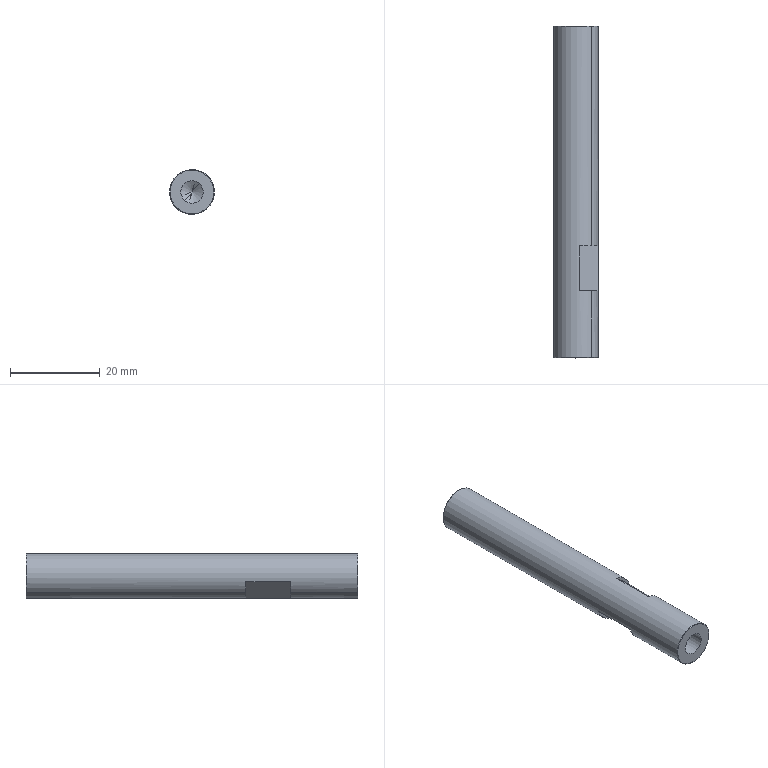Component | SolidWorks | F12529-M5105-2 | 1 solid | 22 faces | box 10 x 74 x 10 mm | volume 5066 mm3 | cone 8 | plane 8 | cylinder 6 | commonest cylinder face diameters 5 x4 10 x2
build123d program:
from build123d import *

# Parameters (mm, degrees)
SKETCH1_R             = 5
EXTRUDE1_DEPTH        = 74
CHAMFER1_SIZE         = 0.1
M6_TAPPED_HOLE1_D     = 5
M6_TAPPED_HOLE1_DEPTH = 17
M6_TAPPED_HOLE1_TIP   = 1.502
M6_TAPPED_HOLE2_D     = 5
M6_TAPPED_HOLE2_DEPTH = 17
M6_TAPPED_HOLE2_TIP   = 1.502
CUT_EXTRUDE2_START    = 4.2
SKETCH6_W             = 12
SKETCH6_H             = 10
CUT_EXTRUDE2_DEPTH    = 10


with BuildPart() as part:
    # Sketch1 → Extrude1 (new body)
    with BuildSketch(Plane(origin=(0, 0, 0), x_dir=(1, 0, 0), z_dir=(0, 1, 0))):
        with Locations(Location((0, 0, 0), (0, 0, 270))):
            Circle(SKETCH1_R)
    extrude(amount=EXTRUDE1_DEPTH)

    # Chamfer1
    chamfer1_edges = [part.edges().sort_by_distance(p)[0] for p in [
        (0, 0, -5),
        (0, 74, -5),
    ]]
    chamfer(chamfer1_edges, length=CHAMFER1_SIZE)

    # M6 Tapped Hole1
    with Locations(Plane(origin=(0, 74, 0), x_dir=(-1, 0, 0), z_dir=(0, 1, 0))):
        with Locations((0, 0)):
            Hole(M6_TAPPED_HOLE1_D / 2, depth=M6_TAPPED_HOLE1_DEPTH)
            with Locations((0, 0, -(M6_TAPPED_HOLE1_DEPTH + M6_TAPPED_HOLE1_TIP / 2))):  # 118° drill point
                Cone(0, M6_TAPPED_HOLE1_D / 2, M6_TAPPED_HOLE1_TIP, mode=Mode.SUBTRACT)

    # M6 Tapped Hole2
    with Locations(Plane.XZ):
        with Locations((0, 0)):
            Hole(M6_TAPPED_HOLE2_D / 2, depth=M6_TAPPED_HOLE2_DEPTH)
            with Locations((0, 0, -(M6_TAPPED_HOLE2_DEPTH + M6_TAPPED_HOLE2_TIP / 2))):  # 118° drill point
                Cone(0, M6_TAPPED_HOLE2_D / 2, M6_TAPPED_HOLE2_TIP, mode=Mode.SUBTRACT)

    # Sketch6 → Cut-Extrude2 (cut)
    with BuildSketch(Plane.XY.offset(CUT_EXTRUDE2_START)):
        with Locations((0, 20)):
            Rectangle(SKETCH6_W, SKETCH6_H)
    cut_extrude2 = extrude(amount=CUT_EXTRUDE2_DEPTH, mode=Mode.SUBTRACT)

    # Mirror1: Cut-Extrude2 across plane
    add(cut_extrude2.mirror(Plane.XY), mode=Mode.SUBTRACT)


solid = part.part

# Placed as in the assembly
solid = solid.moved(Location((-37.5, 201, -10), (180, -42.85, 180)))
STEP:
#1=COLOUR_RGB('',0.7922,0.8196,0.9333);
#2=FILL_AREA_STYLE_COLOUR('',#1);
#3=FILL_AREA_STYLE('',(#2));
#4=SURFACE_STYLE_FILL_AREA(#3);
#5=SURFACE_SIDE_STYLE('',(#4));
#6=SURFACE_STYLE_USAGE(.BOTH.,#5);
#7=PRESENTATION_STYLE_ASSIGNMENT((#6));
#8=CARTESIAN_POINT('',(-1.476,8.642,-0.3937));
#9=VERTEX_POINT('',#8);
#10=CARTESIAN_POINT('',(-1.543,8.583,-0.4659));
#11=VERTEX_POINT('',#10);
#12=CARTESIAN_POINT('',(-1.543,8.583,-0.4659));
#13=DIRECTION('',(-0.5829,-0.515,-0.6284));
#14=VECTOR('',#13,39.37);
#15=LINE('',#12,#14);
#16=EDGE_CURVE('',#9,#11,#15,.T.);
#17=ORIENTED_EDGE('',*,*,#16,.F.);
#18=CARTESIAN_POINT('',(-1.409,8.583,-0.3215));
#19=VERTEX_POINT('',#18);
#20=CARTESIAN_POINT('',(-1.409,8.583,-0.3215));
#21=DIRECTION('',(0.5829,-0.515,0.6284));
#22=VECTOR('',#21,39.37);
#23=LINE('',#20,#22);
#24=EDGE_CURVE('',#9,#19,#23,.T.);
#25=ORIENTED_EDGE('',*,*,#24,.T.);
#26=CARTESIAN_POINT('',(-1.476,8.583,-0.3937));
#27=DIRECTION('',(0.,-1.,0.));
#28=DIRECTION('',(-0.6801,0.,-0.7331));
#29=AXIS2_PLACEMENT_3D('',#26,#27,#28);
#30=CIRCLE('',#29,0.09843);
#31=EDGE_CURVE('',#19,#11,#30,.T.);
#32=ORIENTED_EDGE('',*,*,#31,.T.);
#33=EDGE_LOOP('',(#17,#25,#32));
#34=FACE_OUTER_BOUND('',#33,.T.);
#35=CARTESIAN_POINT('',(-1.476,8.583,-0.3937));
#36=DIRECTION('',(0.,-1.,0.));
#37=DIRECTION('',(-0.6801,0.,-0.7331));
#38=AXIS2_PLACEMENT_3D('',#35,#36,#37);
#39=CONICAL_SURFACE('',#38,0.09843,1.03);
#40=ADVANCED_FACE('',(#34),#39,.F.);
#41=ORIENTED_EDGE('',*,*,#31,.F.);
#42=CARTESIAN_POINT('',(-1.409,7.913,-0.3215));
#43=VERTEX_POINT('',#42);
#44=CARTESIAN_POINT('',(-1.409,7.913,-0.3215));
#45=DIRECTION('',(0.,-1.,0.));
#46=VECTOR('',#45,39.37);
#47=LINE('',#44,#46);
#48=EDGE_CURVE('',#19,#43,#47,.T.);
#49=ORIENTED_EDGE('',*,*,#48,.T.);
#50=CARTESIAN_POINT('',(-1.543,7.913,-0.4659));
#51=VERTEX_POINT('',#50);
#52=CARTESIAN_POINT('',(-1.476,7.913,-0.3937));
#53=DIRECTION('',(0.,-1.,0.));
#54=DIRECTION('',(-0.6801,0.,-0.7331));
#55=AXIS2_PLACEMENT_3D('',#52,#53,#54);
#56=CIRCLE('',#55,0.09843);
#57=EDGE_CURVE('',#43,#51,#56,.T.);
#58=ORIENTED_EDGE('',*,*,#57,.T.);
#59=CARTESIAN_POINT('',(-1.543,7.913,-0.4659));
#60=DIRECTION('',(0.,-1.,0.));
#61=VECTOR('',#60,39.37);
#62=LINE('',#59,#61);
#63=EDGE_CURVE('',#11,#51,#62,.T.);
#64=ORIENTED_EDGE('',*,*,#63,.F.);
#65=EDGE_LOOP('',(#41,#49,#58,#64));
#66=FACE_OUTER_BOUND('',#65,.T.);
#67=CARTESIAN_POINT('',(-1.476,7.913,-0.3937));
#68=DIRECTION('',(0.,-1.,0.));
#69=DIRECTION('',(-0.6801,0.,-0.7331));
#70=AXIS2_PLACEMENT_3D('',#67,#68,#69);
#71=CYLINDRICAL_SURFACE('',#70,0.09843);
#72=ADVANCED_FACE('',(#66),#71,.F.);
#73=CARTESIAN_POINT('',(-1.476,10.098,-0.3937));
#74=VERTEX_POINT('',#73);
#75=CARTESIAN_POINT('',(-1.409,10.157,-0.3215));
#76=VERTEX_POINT('',#75);
#77=CARTESIAN_POINT('',(-1.409,10.157,-0.3215));
#78=DIRECTION('',(0.5829,0.515,0.6284));
#79=VECTOR('',#78,39.37);
#80=LINE('',#77,#79);
#81=EDGE_CURVE('',#74,#76,#80,.T.);
#82=ORIENTED_EDGE('',*,*,#81,.F.);
#83=CARTESIAN_POINT('',(-1.543,10.157,-0.4659));
#84=VERTEX_POINT('',#83);
#85=CARTESIAN_POINT('',(-1.543,10.157,-0.4659));
#86=DIRECTION('',(-0.5829,0.515,-0.6284));
#87=VECTOR('',#86,39.37);
#88=LINE('',#85,#87);
#89=EDGE_CURVE('',#74,#84,#88,.T.);
#90=ORIENTED_EDGE('',*,*,#89,.T.);
#91=CARTESIAN_POINT('',(-1.476,10.157,-0.3937));
#92=DIRECTION('',(0.,1.,0.));
#93=DIRECTION('',(0.6801,0.,0.7331));
#94=AXIS2_PLACEMENT_3D('',#91,#92,#93);
#95=CIRCLE('',#94,0.09843);
#96=EDGE_CURVE('',#84,#76,#95,.T.);
#97=ORIENTED_EDGE('',*,*,#96,.T.);
#98=EDGE_LOOP('',(#82,#90,#97));
#99=FACE_OUTER_BOUND('',#98,.T.);
#100=CARTESIAN_POINT('',(-1.476,10.157,-0.3937));
#101=DIRECTION('',(0.,1.,0.));
#102=DIRECTION('',(0.6801,0.,0.7331));
#103=AXIS2_PLACEMENT_3D('',#100,#101,#102);
#104=CONICAL_SURFACE('',#103,0.09843,1.03);
#105=ADVANCED_FACE('',(#99),#104,.F.);
#106=ORIENTED_EDGE('',*,*,#96,.F.);
#107=CARTESIAN_POINT('',(-1.543,10.827,-0.4659));
#108=VERTEX_POINT('',#107);
#109=CARTESIAN_POINT('',(-1.543,10.827,-0.4659));
#110=DIRECTION('',(0.,1.,0.));
#111=VECTOR('',#110,39.37);
#112=LINE('',#109,#111);
#113=EDGE_CURVE('',#84,#108,#112,.T.);
#114=ORIENTED_EDGE('',*,*,#113,.T.);
#115=CARTESIAN_POINT('',(-1.409,10.827,-0.3215));
#116=VERTEX_POINT('',#115);
#117=CARTESIAN_POINT('',(-1.476,10.827,-0.3937));
#118=DIRECTION('',(0.,1.,0.));
#119=DIRECTION('',(0.6801,0.,0.7331));
#120=AXIS2_PLACEMENT_3D('',#117,#118,#119);
#121=CIRCLE('',#120,0.09843);
#122=EDGE_CURVE('',#108,#116,#121,.T.);
#123=ORIENTED_EDGE('',*,*,#122,.T.);
#124=CARTESIAN_POINT('',(-1.409,10.827,-0.3215));
#125=DIRECTION('',(0.,1.,0.));
#126=VECTOR('',#125,39.37);
#127=LINE('',#124,#126);
#128=EDGE_CURVE('',#76,#116,#127,.T.);
#129=ORIENTED_EDGE('',*,*,#128,.F.);
#130=EDGE_LOOP('',(#106,#114,#123,#129));
#131=FACE_OUTER_BOUND('',#130,.T.);
#132=CARTESIAN_POINT('',(-1.476,10.827,-0.3937));
#133=DIRECTION('',(0.,1.,0.));
#134=DIRECTION('',(0.6801,0.,0.7331));
#135=AXIS2_PLACEMENT_3D('',#132,#133,#134);
#136=CYLINDRICAL_SURFACE('',#135,0.09843);
#137=ADVANCED_FACE('',(#131),#136,.F.);
#138=CARTESIAN_POINT('',(-1.345,10.827,-0.2523));
#139=VERTEX_POINT('',#138);
#140=CARTESIAN_POINT('',(-1.608,10.827,-0.5351));
#141=VERTEX_POINT('',#140);
#142=CARTESIAN_POINT('',(-1.476,10.827,-0.3937));
#143=DIRECTION('',(0.,1.,0.));
#144=DIRECTION('',(0.6801,0.,0.7331));
#145=AXIS2_PLACEMENT_3D('',#142,#143,#144);
#146=CIRCLE('',#145,0.1929);
#147=EDGE_CURVE('',#139,#141,#146,.T.);
#148=ORIENTED_EDGE('',*,*,#147,.F.);
#149=CARTESIAN_POINT('',(-1.343,10.823,-0.2494));
#150=VERTEX_POINT('',#149);
#151=CARTESIAN_POINT('',(-1.345,10.827,-0.2523));
#152=DIRECTION('',(0.4809,-0.7071,0.5184));
#153=VECTOR('',#152,39.37);
#154=LINE('',#151,#153);
#155=EDGE_CURVE('',#139,#150,#154,.T.);
#156=ORIENTED_EDGE('',*,*,#155,.T.);
#157=CARTESIAN_POINT('',(-1.61,10.823,-0.538));
#158=VERTEX_POINT('',#157);
#159=CARTESIAN_POINT('',(-1.476,10.823,-0.3937));
#160=DIRECTION('',(0.,-1.,0.));
#161=DIRECTION('',(0.6801,0.,0.7331));
#162=AXIS2_PLACEMENT_3D('',#159,#160,#161);
#163=CIRCLE('',#162,0.1969);
#164=EDGE_CURVE('',#158,#150,#163,.T.);
#165=ORIENTED_EDGE('',*,*,#164,.F.);
#166=CARTESIAN_POINT('',(-1.608,10.827,-0.5351));
#167=DIRECTION('',(-0.4809,-0.7071,-0.5184));
#168=VECTOR('',#167,39.37);
#169=LINE('',#166,#168);
#170=EDGE_CURVE('',#141,#158,#169,.T.);
#171=ORIENTED_EDGE('',*,*,#170,.F.);
#172=EDGE_LOOP('',(#148,#156,#165,#171));
#173=FACE_OUTER_BOUND('',#172,.T.);
#174=CARTESIAN_POINT('',(-1.476,10.827,-0.3937));
#175=DIRECTION('',(0.,-1.,0.));
#176=DIRECTION('',(-0.6801,0.,-0.7331));
#177=AXIS2_PLACEMENT_3D('',#174,#175,#176);
#178=CONICAL_SURFACE('',#177,0.1929,0.7854);
#179=ADVANCED_FACE('',(#173),#178,.T.);
#180=CARTESIAN_POINT('',(-1.608,7.913,-0.5351));
#181=VERTEX_POINT('',#180);
#182=CARTESIAN_POINT('',(-1.345,7.913,-0.2523));
#183=VERTEX_POINT('',#182);
#184=CARTESIAN_POINT('',(-1.476,7.913,-0.3937));
#185=DIRECTION('',(0.,-1.,0.));
#186=DIRECTION('',(0.6801,0.,0.7331));
#187=AXIS2_PLACEMENT_3D('',#184,#185,#186);
#188=CIRCLE('',#187,0.1929);
#189=EDGE_CURVE('',#181,#183,#188,.T.);
#190=ORIENTED_EDGE('',*,*,#189,.F.);
#191=CARTESIAN_POINT('',(-1.61,7.917,-0.538));
#192=VERTEX_POINT('',#191);
#193=CARTESIAN_POINT('',(-1.61,7.917,-0.538));
#194=DIRECTION('',(-0.4809,0.7071,-0.5184));
#195=VECTOR('',#194,39.37);
#196=LINE('',#193,#195);
#197=EDGE_CURVE('',#181,#192,#196,.T.);
#198=ORIENTED_EDGE('',*,*,#197,.T.);
#199=CARTESIAN_POINT('',(-1.343,7.917,-0.2494));
#200=VERTEX_POINT('',#199);
#201=CARTESIAN_POINT('',(-1.476,7.917,-0.3937));
#202=DIRECTION('',(0.,1.,0.));
#203=DIRECTION('',(0.6801,0.,0.7331));
#204=AXIS2_PLACEMENT_3D('',#201,#202,#203);
#205=CIRCLE('',#204,0.1969);
#206=EDGE_CURVE('',#200,#192,#205,.T.);
#207=ORIENTED_EDGE('',*,*,#206,.F.);
#208=CARTESIAN_POINT('',(-1.343,7.917,-0.2494));
#209=DIRECTION('',(0.4809,0.7071,0.5184));
#210=VECTOR('',#209,39.37);
#211=LINE('',#208,#210);
#212=EDGE_CURVE('',#183,#200,#211,.T.);
#213=ORIENTED_EDGE('',*,*,#212,.F.);
#214=EDGE_LOOP('',(#190,#198,#207,#213));
#215=FACE_OUTER_BOUND('',#214,.T.);
#216=CARTESIAN_POINT('',(-1.476,7.917,-0.3937));
#217=DIRECTION('',(0.,1.,0.));
#218=DIRECTION('',(0.6801,0.,0.7331));
#219=AXIS2_PLACEMENT_3D('',#216,#217,#218);
#220=CONICAL_SURFACE('',#219,0.1969,0.7854);
#221=ADVANCED_FACE('',(#215),#220,.T.);
#222=ORIENTED_EDGE('',*,*,#164,.T.);
#223=CARTESIAN_POINT('',(-1.343,8.898,-0.2494));
#224=VERTEX_POINT('',#223);
#225=CARTESIAN_POINT('',(-1.343,10.827,-0.2494));
#226=DIRECTION('',(0.,-1.,0.));
#227=VECTOR('',#226,39.37);
#228=LINE('',#225,#227);
#229=EDGE_CURVE('',#150,#224,#228,.T.);
#230=ORIENTED_EDGE('',*,*,#229,.T.);
#231=CARTESIAN_POINT('',(-1.286,8.898,-0.3451));
#232=VERTEX_POINT('',#231);
#233=CARTESIAN_POINT('',(-1.476,8.898,-0.3937));
#234=DIRECTION('',(0.,-1.,0.));
#235=DIRECTION('',(-0.6801,0.,-0.7331));
#236=AXIS2_PLACEMENT_3D('',#233,#234,#235);
#237=CIRCLE('',#236,0.1969);
#238=EDGE_CURVE('',#232,#224,#237,.T.);
#239=ORIENTED_EDGE('',*,*,#238,.F.);
#240=CARTESIAN_POINT('',(-1.286,8.504,-0.3451));
#241=VERTEX_POINT('',#240);
#242=CARTESIAN_POINT('',(-1.286,10.827,-0.3451));
#243=DIRECTION('',(0.,1.,0.));
#244=VECTOR('',#243,39.37);
#245=LINE('',#242,#244);
#246=EDGE_CURVE('',#241,#232,#245,.T.);
#247=ORIENTED_EDGE('',*,*,#246,.F.);
#248=CARTESIAN_POINT('',(-1.343,8.504,-0.2494));
#249=VERTEX_POINT('',#248);
#250=CARTESIAN_POINT('',(-1.476,8.504,-0.3937));
#251=DIRECTION('',(0.,1.,0.));
#252=DIRECTION('',(0.6801,0.,0.7331));
#253=AXIS2_PLACEMENT_3D('',#250,#251,#252);
#254=CIRCLE('',#253,0.1969);
#255=EDGE_CURVE('',#249,#241,#254,.T.);
#256=ORIENTED_EDGE('',*,*,#255,.F.);
#257=CARTESIAN_POINT('',(-1.343,10.827,-0.2494));
#258=DIRECTION('',(0.,-1.,0.));
#259=VECTOR('',#258,39.37);
#260=LINE('',#257,#259);
#261=EDGE_CURVE('',#249,#200,#260,.T.);
#262=ORIENTED_EDGE('',*,*,#261,.T.);
#263=ORIENTED_EDGE('',*,*,#206,.T.);
#264=CARTESIAN_POINT('',(-1.61,8.504,-0.538));
#265=VERTEX_POINT('',#264);
#266=CARTESIAN_POINT('',(-1.61,10.827,-0.538));
#267=DIRECTION('',(0.,-1.,0.));
#268=VECTOR('',#267,39.37);
#269=LINE('',#266,#268);
#270=EDGE_CURVE('',#265,#192,#269,.T.);
#271=ORIENTED_EDGE('',*,*,#270,.F.);
#272=CARTESIAN_POINT('',(-1.511,8.504,-0.5876));
#273=VERTEX_POINT('',#272);
#274=CARTESIAN_POINT('',(-1.476,8.504,-0.3937));
#275=DIRECTION('',(0.,-1.,0.));
#276=DIRECTION('',(-0.6801,0.,-0.7331));
#277=AXIS2_PLACEMENT_3D('',#274,#275,#276);
#278=CIRCLE('',#277,0.1969);
#279=EDGE_CURVE('',#265,#273,#278,.T.);
#280=ORIENTED_EDGE('',*,*,#279,.T.);
#281=CARTESIAN_POINT('',(-1.511,8.898,-0.5876));
#282=VERTEX_POINT('',#281);
#283=CARTESIAN_POINT('',(-1.511,10.827,-0.5876));
#284=DIRECTION('',(0.,-1.,0.));
#285=VECTOR('',#284,39.37);
#286=LINE('',#283,#285);
#287=EDGE_CURVE('',#282,#273,#286,.T.);
#288=ORIENTED_EDGE('',*,*,#287,.F.);
#289=CARTESIAN_POINT('',(-1.61,8.898,-0.538));
#290=VERTEX_POINT('',#289);
#291=CARTESIAN_POINT('',(-1.476,8.898,-0.3937));
#292=DIRECTION('',(0.,1.,0.));
#293=DIRECTION('',(0.6801,0.,0.7331));
#294=AXIS2_PLACEMENT_3D('',#291,#292,#293);
#295=CIRCLE('',#294,0.1969);
#296=EDGE_CURVE('',#282,#290,#295,.T.);
#297=ORIENTED_EDGE('',*,*,#296,.T.);
#298=CARTESIAN_POINT('',(-1.61,10.827,-0.538));
#299=DIRECTION('',(0.,-1.,0.));
#300=VECTOR('',#299,39.37);
#301=LINE('',#298,#300);
#302=EDGE_CURVE('',#158,#290,#301,.T.);
#303=ORIENTED_EDGE('',*,*,#302,.F.);
#304=EDGE_LOOP('',(#222,#230,#239,#247,#256,#262,#263,#271,#280,#288,#297,#303));
#305=FACE_OUTER_BOUND('',#304,.T.);
#306=CARTESIAN_POINT('',(-1.476,10.827,-0.3937));
#307=DIRECTION('',(0.,-1.,0.));
#308=DIRECTION('',(-0.6801,0.,-0.7331));
#309=AXIS2_PLACEMENT_3D('',#306,#307,#308);
#310=CYLINDRICAL_SURFACE('',#309,0.1969);
#311=ADVANCED_FACE('',(#305),#310,.T.);
#312=ORIENTED_EDGE('',*,*,#229,.F.);
#313=CARTESIAN_POINT('',(-1.476,10.823,-0.3937));
#314=DIRECTION('',(0.,-1.,0.));
#315=DIRECTION('',(0.6801,0.,0.7331));
#316=AXIS2_PLACEMENT_3D('',#313,#314,#315);
#317=CIRCLE('',#316,0.1969);
#318=EDGE_CURVE('',#150,#158,#317,.T.);
#319=ORIENTED_EDGE('',*,*,#318,.T.);
#320=ORIENTED_EDGE('',*,*,#302,.T.);
#321=CARTESIAN_POINT('',(-1.667,8.898,-0.4423));
#322=VERTEX_POINT('',#321);
#323=CARTESIAN_POINT('',(-1.476,8.898,-0.3937));
#324=DIRECTION('',(0.,1.,0.));
#325=DIRECTION('',(0.6801,0.,0.7331));
#326=AXIS2_PLACEMENT_3D('',#323,#324,#325);
#327=CIRCLE('',#326,0.1969);
#328=EDGE_CURVE('',#290,#322,#327,.T.);
#329=ORIENTED_EDGE('',*,*,#328,.T.);
#330=CARTESIAN_POINT('',(-1.667,8.504,-0.4423));
#331=VERTEX_POINT('',#330);
#332=CARTESIAN_POINT('',(-1.667,10.827,-0.4423));
#333=DIRECTION('',(0.,1.,0.));
#334=VECTOR('',#333,39.37);
#335=LINE('',#332,#334);
#336=EDGE_CURVE('',#331,#322,#335,.T.);
#337=ORIENTED_EDGE('',*,*,#336,.F.);
#338=CARTESIAN_POINT('',(-1.476,8.504,-0.3937));
#339=DIRECTION('',(0.,-1.,0.));
#340=DIRECTION('',(-0.6801,0.,-0.7331));
#341=AXIS2_PLACEMENT_3D('',#338,#339,#340);
#342=CIRCLE('',#341,0.1969);
#343=EDGE_CURVE('',#331,#265,#342,.T.);
#344=ORIENTED_EDGE('',*,*,#343,.T.);
#345=ORIENTED_EDGE('',*,*,#270,.T.);
#346=CARTESIAN_POINT('',(-1.476,7.917,-0.3937));
#347=DIRECTION('',(0.,1.,0.));
#348=DIRECTION('',(0.6801,0.,0.7331));
#349=AXIS2_PLACEMENT_3D('',#346,#347,#348);
#350=CIRCLE('',#349,0.1969);
#351=EDGE_CURVE('',#192,#200,#350,.T.);
#352=ORIENTED_EDGE('',*,*,#351,.T.);
#353=ORIENTED_EDGE('',*,*,#261,.F.);
#354=CARTESIAN_POINT('',(-1.442,8.504,-0.1998));
#355=VERTEX_POINT('',#354);
#356=CARTESIAN_POINT('',(-1.476,8.504,-0.3937));
#357=DIRECTION('',(0.,1.,0.));
#358=DIRECTION('',(0.6801,0.,0.7331));
#359=AXIS2_PLACEMENT_3D('',#356,#357,#358);
#360=CIRCLE('',#359,0.1969);
#361=EDGE_CURVE('',#355,#249,#360,.T.);
#362=ORIENTED_EDGE('',*,*,#361,.F.);
#363=CARTESIAN_POINT('',(-1.442,8.898,-0.1998));
#364=VERTEX_POINT('',#363);
#365=CARTESIAN_POINT('',(-1.442,10.827,-0.1998));
#366=DIRECTION('',(0.,-1.,0.));
#367=VECTOR('',#366,39.37);
#368=LINE('',#365,#367);
#369=EDGE_CURVE('',#364,#355,#368,.T.);
#370=ORIENTED_EDGE('',*,*,#369,.F.);
#371=CARTESIAN_POINT('',(-1.476,8.898,-0.3937));
#372=DIRECTION('',(0.,-1.,0.));
#373=DIRECTION('',(-0.6801,0.,-0.7331));
#374=AXIS2_PLACEMENT_3D('',#371,#372,#373);
#375=CIRCLE('',#374,0.1969);
#376=EDGE_CURVE('',#224,#364,#375,.T.);
#377=ORIENTED_EDGE('',*,*,#376,.F.);
#378=EDGE_LOOP('',(#312,#319,#320,#329,#337,#344,#345,#352,#353,#362,#370,#377));
#379=FACE_OUTER_BOUND('',#378,.T.);
#380=CARTESIAN_POINT('',(-1.476,10.827,-0.3937));
#381=DIRECTION('',(0.,-1.,0.));
#382=DIRECTION('',(-0.6801,0.,-0.7331));
#383=AXIS2_PLACEMENT_3D('',#380,#381,#382);
#384=CYLINDRICAL_SURFACE('',#383,0.1969);
#385=ADVANCED_FACE('',(#379),#384,.T.);
#386=CARTESIAN_POINT('',(-1.476,10.827,-0.3937));
#387=DIRECTION('',(0.,1.,0.));
#388=DIRECTION('',(0.6801,0.,0.7331));
#389=AXIS2_PLACEMENT_3D('',#386,#387,#388);
#390=CIRCLE('',#389,0.09843);
#391=EDGE_CURVE('',#116,#108,#390,.T.);
#392=ORIENTED_EDGE('',*,*,#391,.F.);
#393=ORIENTED_EDGE('',*,*,#122,.F.);
#394=EDGE_LOOP('',(#392,#393));
#395=FACE_BOUND('',#394,.T.);
#396=CARTESIAN_POINT('',(-1.476,10.827,-0.3937));
#397=DIRECTION('',(0.,1.,0.));
#398=DIRECTION('',(0.6801,0.,0.7331));
#399=AXIS2_PLACEMENT_3D('',#396,#397,#398);
#400=CIRCLE('',#399,0.1929);
#401=EDGE_CURVE('',#141,#139,#400,.T.);
#402=ORIENTED_EDGE('',*,*,#401,.T.);
#403=ORIENTED_EDGE('',*,*,#147,.T.);
#404=EDGE_LOOP('',(#402,#403));
#405=FACE_OUTER_BOUND('',#404,.T.);
#406=CARTESIAN_POINT('',(-1.476,10.827,-0.3937));
#407=DIRECTION('',(0.,1.,0.));
#408=DIRECTION('',(0.6801,0.,0.7331));
#409=AXIS2_PLACEMENT_3D('',#406,#407,#408);
#410=PLANE('',#409);
#411=ADVANCED_FACE('',(#395,#405),#410,.T.);
#412=CARTESIAN_POINT('',(-1.476,7.913,-0.3937));
#413=DIRECTION('',(0.,-1.,0.));
#414=DIRECTION('',(-0.6801,0.,-0.7331));
#415=AXIS2_PLACEMENT_3D('',#412,#413,#414);
#416=CIRCLE('',#415,0.09843);
#417=EDGE_CURVE('',#51,#43,#416,.T.);
#418=ORIENTED_EDGE('',*,*,#417,.F.);
#419=ORIENTED_EDGE('',*,*,#57,.F.);
#420=EDGE_LOOP('',(#418,#419));
#421=FACE_BOUND('',#420,.T.);
#422=CARTESIAN_POINT('',(-1.476,7.913,-0.3937));
#423=DIRECTION('',(0.,-1.,0.));
#424=DIRECTION('',(0.6801,0.,0.7331));
#425=AXIS2_PLACEMENT_3D('',#422,#423,#424);
#426=CIRCLE('',#425,0.1929);
#427=EDGE_CURVE('',#183,#181,#426,.T.);
#428=ORIENTED_EDGE('',*,*,#427,.T.);
#429=ORIENTED_EDGE('',*,*,#189,.T.);
#430=EDGE_LOOP('',(#428,#429));
#431=FACE_OUTER_BOUND('',#430,.T.);
#432=CARTESIAN_POINT('',(-1.476,7.913,-0.3937));
#433=DIRECTION('',(0.,1.,0.));
#434=DIRECTION('',(0.6801,0.,0.7331));
#435=AXIS2_PLACEMENT_3D('',#432,#433,#434);
#436=PLANE('',#435);
#437=ADVANCED_FACE('',(#421,#431),#436,.F.);
#438=ORIENTED_EDGE('',*,*,#197,.F.);
#439=ORIENTED_EDGE('',*,*,#427,.F.);
#440=ORIENTED_EDGE('',*,*,#212,.T.);
#441=ORIENTED_EDGE('',*,*,#351,.F.);
#442=EDGE_LOOP('',(#438,#439,#440,#441));
#443=FACE_OUTER_BOUND('',#442,.T.);
#444=CARTESIAN_POINT('',(-1.476,7.917,-0.3937));
#445=DIRECTION('',(0.,1.,0.));
#446=DIRECTION('',(0.6801,0.,0.7331));
#447=AXIS2_PLACEMENT_3D('',#444,#445,#446);
#448=CONICAL_SURFACE('',#447,0.1969,0.7854);
#449=ADVANCED_FACE('',(#443),#448,.T.);
#450=ORIENTED_EDGE('',*,*,#155,.F.);
#451=ORIENTED_EDGE('',*,*,#401,.F.);
#452=ORIENTED_EDGE('',*,*,#170,.T.);
#453=ORIENTED_EDGE('',*,*,#318,.F.);
#454=EDGE_LOOP('',(#450,#451,#452,#453));
#455=FACE_OUTER_BOUND('',#454,.T.);
#456=CARTESIAN_POINT('',(-1.476,10.827,-0.3937));
#457=DIRECTION('',(0.,-1.,0.));
#458=DIRECTION('',(-0.6801,0.,-0.7331));
#459=AXIS2_PLACEMENT_3D('',#456,#457,#458);
#460=CONICAL_SURFACE('',#459,0.1929,0.7854);
#461=ADVANCED_FACE('',(#455),#460,.T.);
#462=ORIENTED_EDGE('',*,*,#113,.F.);
#463=CARTESIAN_POINT('',(-1.476,10.157,-0.3937));
#464=DIRECTION('',(0.,1.,0.));
#465=DIRECTION('',(0.6801,0.,0.7331));
#466=AXIS2_PLACEMENT_3D('',#463,#464,#465);
#467=CIRCLE('',#466,0.09843);
#468=EDGE_CURVE('',#76,#84,#467,.T.);
#469=ORIENTED_EDGE('',*,*,#468,.F.);
#470=ORIENTED_EDGE('',*,*,#128,.T.);
#471=ORIENTED_EDGE('',*,*,#391,.T.);
#472=EDGE_LOOP('',(#462,#469,#470,#471));
#473=FACE_OUTER_BOUND('',#472,.T.);
#474=CARTESIAN_POINT('',(-1.476,10.827,-0.3937));
#475=DIRECTION('',(0.,1.,0.));
#476=DIRECTION('',(0.6801,0.,0.7331));
#477=AXIS2_PLACEMENT_3D('',#474,#475,#476);
#478=CYLINDRICAL_SURFACE('',#477,0.09843);
#479=ADVANCED_FACE('',(#473),#478,.F.);
#480=ORIENTED_EDGE('',*,*,#89,.F.);
#481=ORIENTED_EDGE('',*,*,#81,.T.);
#482=ORIENTED_EDGE('',*,*,#468,.T.);
#483=EDGE_LOOP('',(#480,#481,#482));
#484=FACE_OUTER_BOUND('',#483,.T.);
#485=CARTESIAN_POINT('',(-1.476,10.157,-0.3937));
#486=DIRECTION('',(0.,1.,0.));
#487=DIRECTION('',(0.6801,0.,0.7331));
#488=AXIS2_PLACEMENT_3D('',#485,#486,#487);
#489=CONICAL_SURFACE('',#488,0.09843,1.03);
#490=ADVANCED_FACE('',(#484),#489,.F.);
#491=ORIENTED_EDGE('',*,*,#48,.F.);
#492=CARTESIAN_POINT('',(-1.476,8.583,-0.3937));
#493=DIRECTION('',(0.,-1.,0.));
#494=DIRECTION('',(-0.6801,0.,-0.7331));
#495=AXIS2_PLACEMENT_3D('',#492,#493,#494);
#496=CIRCLE('',#495,0.09843);
#497=EDGE_CURVE('',#11,#19,#496,.T.);
#498=ORIENTED_EDGE('',*,*,#497,.F.);
#499=ORIENTED_EDGE('',*,*,#63,.T.);
#500=ORIENTED_EDGE('',*,*,#417,.T.);
#501=EDGE_LOOP('',(#491,#498,#499,#500));
#502=FACE_OUTER_BOUND('',#501,.T.);
#503=CARTESIAN_POINT('',(-1.476,7.913,-0.3937));
#504=DIRECTION('',(0.,-1.,0.));
#505=DIRECTION('',(-0.6801,0.,-0.7331));
#506=AXIS2_PLACEMENT_3D('',#503,#504,#505);
#507=CYLINDRICAL_SURFACE('',#506,0.09843);
#508=ADVANCED_FACE('',(#502),#507,.F.);
#509=ORIENTED_EDGE('',*,*,#24,.F.);
#510=ORIENTED_EDGE('',*,*,#16,.T.);
#511=ORIENTED_EDGE('',*,*,#497,.T.);
#512=EDGE_LOOP('',(#509,#510,#511));
#513=FACE_OUTER_BOUND('',#512,.T.);
#514=CARTESIAN_POINT('',(-1.476,8.583,-0.3937));
#515=DIRECTION('',(0.,-1.,0.));
#516=DIRECTION('',(-0.6801,0.,-0.7331));
#517=AXIS2_PLACEMENT_3D('',#514,#515,#516);
#518=CONICAL_SURFACE('',#517,0.09843,1.03);
#519=ADVANCED_FACE('',(#513),#518,.F.);
#520=ORIENTED_EDGE('',*,*,#361,.T.);
#521=ORIENTED_EDGE('',*,*,#255,.T.);
#522=CARTESIAN_POINT('',(-1.537,8.504,-0.1118));
#523=DIRECTION('',(0.7331,0.,-0.6801));
#524=VECTOR('',#523,39.37);
#525=LINE('',#522,#524);
#526=EDGE_CURVE('',#355,#241,#525,.T.);
#527=ORIENTED_EDGE('',*,*,#526,.F.);
#528=EDGE_LOOP('',(#520,#521,#527));
#529=FACE_OUTER_BOUND('',#528,.T.);
#530=CARTESIAN_POINT('',(-1.269,8.504,0.1768));
#531=DIRECTION('',(0.,1.,0.));
#532=DIRECTION('',(0.6801,0.,0.7331));
#533=AXIS2_PLACEMENT_3D('',#530,#531,#532);
#534=PLANE('',#533);
#535=ADVANCED_FACE('',(#529),#534,.T.);
#536=ORIENTED_EDGE('',*,*,#238,.T.);
#537=ORIENTED_EDGE('',*,*,#376,.T.);
#538=CARTESIAN_POINT('',(-1.537,8.898,-0.1118));
#539=DIRECTION('',(-0.7331,0.,0.6801));
#540=VECTOR('',#539,39.37);
#541=LINE('',#538,#540);
#542=EDGE_CURVE('',#232,#364,#541,.T.);
#543=ORIENTED_EDGE('',*,*,#542,.F.);
#544=EDGE_LOOP('',(#536,#537,#543));
#545=FACE_OUTER_BOUND('',#544,.T.);
#546=CARTESIAN_POINT('',(-1.269,8.898,0.1768));
#547=DIRECTION('',(0.,-1.,0.));
#548=DIRECTION('',(-0.6801,0.,-0.7331));
#549=AXIS2_PLACEMENT_3D('',#546,#547,#548);
#550=PLANE('',#549);
#551=ADVANCED_FACE('',(#545),#550,.T.);
#552=ORIENTED_EDGE('',*,*,#369,.T.);
#553=ORIENTED_EDGE('',*,*,#526,.T.);
#554=ORIENTED_EDGE('',*,*,#246,.T.);
#555=ORIENTED_EDGE('',*,*,#542,.T.);
#556=EDGE_LOOP('',(#552,#553,#554,#555));
#557=FACE_OUTER_BOUND('',#556,.T.);
#558=CARTESIAN_POINT('',(-1.537,8.504,-0.1118));
#559=DIRECTION('',(0.6801,0.,0.7331));
#560=DIRECTION('',(0.7331,0.,-0.6801));
#561=AXIS2_PLACEMENT_3D('',#558,#559,#560);
#562=PLANE('',#561);
#563=ADVANCED_FACE('',(#557),#562,.T.);
#564=CARTESIAN_POINT('',(-1.762,8.898,-0.3543));
#565=DIRECTION('',(-0.7331,0.,0.6801));
#566=VECTOR('',#565,39.37);
#567=LINE('',#564,#566);
#568=EDGE_CURVE('',#282,#322,#567,.T.);
#569=ORIENTED_EDGE('',*,*,#568,.T.);
#570=ORIENTED_EDGE('',*,*,#328,.F.);
#571=ORIENTED_EDGE('',*,*,#296,.F.);
#572=EDGE_LOOP('',(#569,#570,#571));
#573=FACE_OUTER_BOUND('',#572,.T.);
#574=CARTESIAN_POINT('',(-2.03,8.898,-0.6429));
#575=DIRECTION('',(0.,1.,0.));
#576=DIRECTION('',(0.6801,0.,0.7331));
#577=AXIS2_PLACEMENT_3D('',#574,#575,#576);
#578=PLANE('',#577);
#579=ADVANCED_FACE('',(#573),#578,.F.);
#580=CARTESIAN_POINT('',(-1.762,8.504,-0.3543));
#581=DIRECTION('',(0.7331,0.,-0.6801));
#582=VECTOR('',#581,39.37);
#583=LINE('',#580,#582);
#584=EDGE_CURVE('',#331,#273,#583,.T.);
#585=ORIENTED_EDGE('',*,*,#584,.T.);
#586=ORIENTED_EDGE('',*,*,#279,.F.);
#587=ORIENTED_EDGE('',*,*,#343,.F.);
#588=EDGE_LOOP('',(#585,#586,#587));
#589=FACE_OUTER_BOUND('',#588,.T.);
#590=CARTESIAN_POINT('',(-2.03,8.504,-0.6429));
#591=DIRECTION('',(0.,-1.,0.));
#592=DIRECTION('',(-0.6801,0.,-0.7331));
#593=AXIS2_PLACEMENT_3D('',#590,#591,#592);
#594=PLANE('',#593);
#595=ADVANCED_FACE('',(#589),#594,.F.);
#596=ORIENTED_EDGE('',*,*,#287,.T.);
#597=ORIENTED_EDGE('',*,*,#584,.F.);
#598=ORIENTED_EDGE('',*,*,#336,.T.);
#599=ORIENTED_EDGE('',*,*,#568,.F.);
#600=EDGE_LOOP('',(#596,#597,#598,#599));
#601=FACE_OUTER_BOUND('',#600,.T.);
#602=CARTESIAN_POINT('',(-1.762,8.504,-0.3543));
#603=DIRECTION('',(-0.6801,0.,-0.7331));
#604=DIRECTION('',(0.7331,0.,-0.6801));
#605=AXIS2_PLACEMENT_3D('',#602,#603,#604);
#606=PLANE('',#605);
#607=ADVANCED_FACE('',(#601),#606,.T.);
#608=CLOSED_SHELL('',(#40,#72,#105,#137,#179,#221,#311,#385,#411,#437,#449,#461,#479,#490,#508,#519,#535,#551,#563,#579,#595,#607));
#609=MANIFOLD_SOLID_BREP('',#608);
#610=STYLED_ITEM('',(#7),#609);
#611=(LENGTH_UNIT()NAMED_UNIT(*)SI_UNIT($,.METRE.));
#612=LENGTH_MEASURE_WITH_UNIT(LENGTH_MEASURE(0.0254),#611);
#613=DIMENSIONAL_EXPONENTS(1.,0.,0.,0.,0.,0.,0.);
#614=(CONVERSION_BASED_UNIT('',#612)LENGTH_UNIT()NAMED_UNIT(#613));
#615=UNCERTAINTY_MEASURE_WITH_UNIT(LENGTH_MEASURE(0.00001),#614,'','');
#616=(NAMED_UNIT(*)PLANE_ANGLE_UNIT()SI_UNIT($,.RADIAN.));
#617=(NAMED_UNIT(*)SI_UNIT($,.STERADIAN.)SOLID_ANGLE_UNIT());
#618=(GEOMETRIC_REPRESENTATION_CONTEXT(3)GLOBAL_UNCERTAINTY_ASSIGNED_CONTEXT((#615))GLOBAL_UNIT_ASSIGNED_CONTEXT((#614,#616,#617))REPRESENTATION_CONTEXT('',''));
#619=MECHANICAL_DESIGN_GEOMETRIC_PRESENTATION_REPRESENTATION('',(#610),#618);
#620=CARTESIAN_POINT('',(0.,0.,0.));
#621=DIRECTION('',(0.,0.,1.));
#622=DIRECTION('',(1.,0.,0.));
#623=AXIS2_PLACEMENT_3D('',#620,#621,#622);
#624=(LENGTH_UNIT()NAMED_UNIT(*)SI_UNIT($,.METRE.));
#625=LENGTH_MEASURE_WITH_UNIT(LENGTH_MEASURE(0.0254),#624);
#626=DIMENSIONAL_EXPONENTS(1.,0.,0.,0.,0.,0.,0.);
#627=(CONVERSION_BASED_UNIT('',#625)LENGTH_UNIT()NAMED_UNIT(#626));
#628=UNCERTAINTY_MEASURE_WITH_UNIT(LENGTH_MEASURE(0.00001),#627,'','');
#629=(NAMED_UNIT(*)PLANE_ANGLE_UNIT()SI_UNIT($,.RADIAN.));
#630=(NAMED_UNIT(*)SI_UNIT($,.STERADIAN.)SOLID_ANGLE_UNIT());
#631=(GEOMETRIC_REPRESENTATION_CONTEXT(3)GLOBAL_UNCERTAINTY_ASSIGNED_CONTEXT((#628))GLOBAL_UNIT_ASSIGNED_CONTEXT((#627,#629,#630))REPRESENTATION_CONTEXT('',''));
#632=ADVANCED_BREP_SHAPE_REPRESENTATION('',(#609,#623),#631);
#633=PRESENTATION_LAYER_ASSIGNMENT('','',(#610));